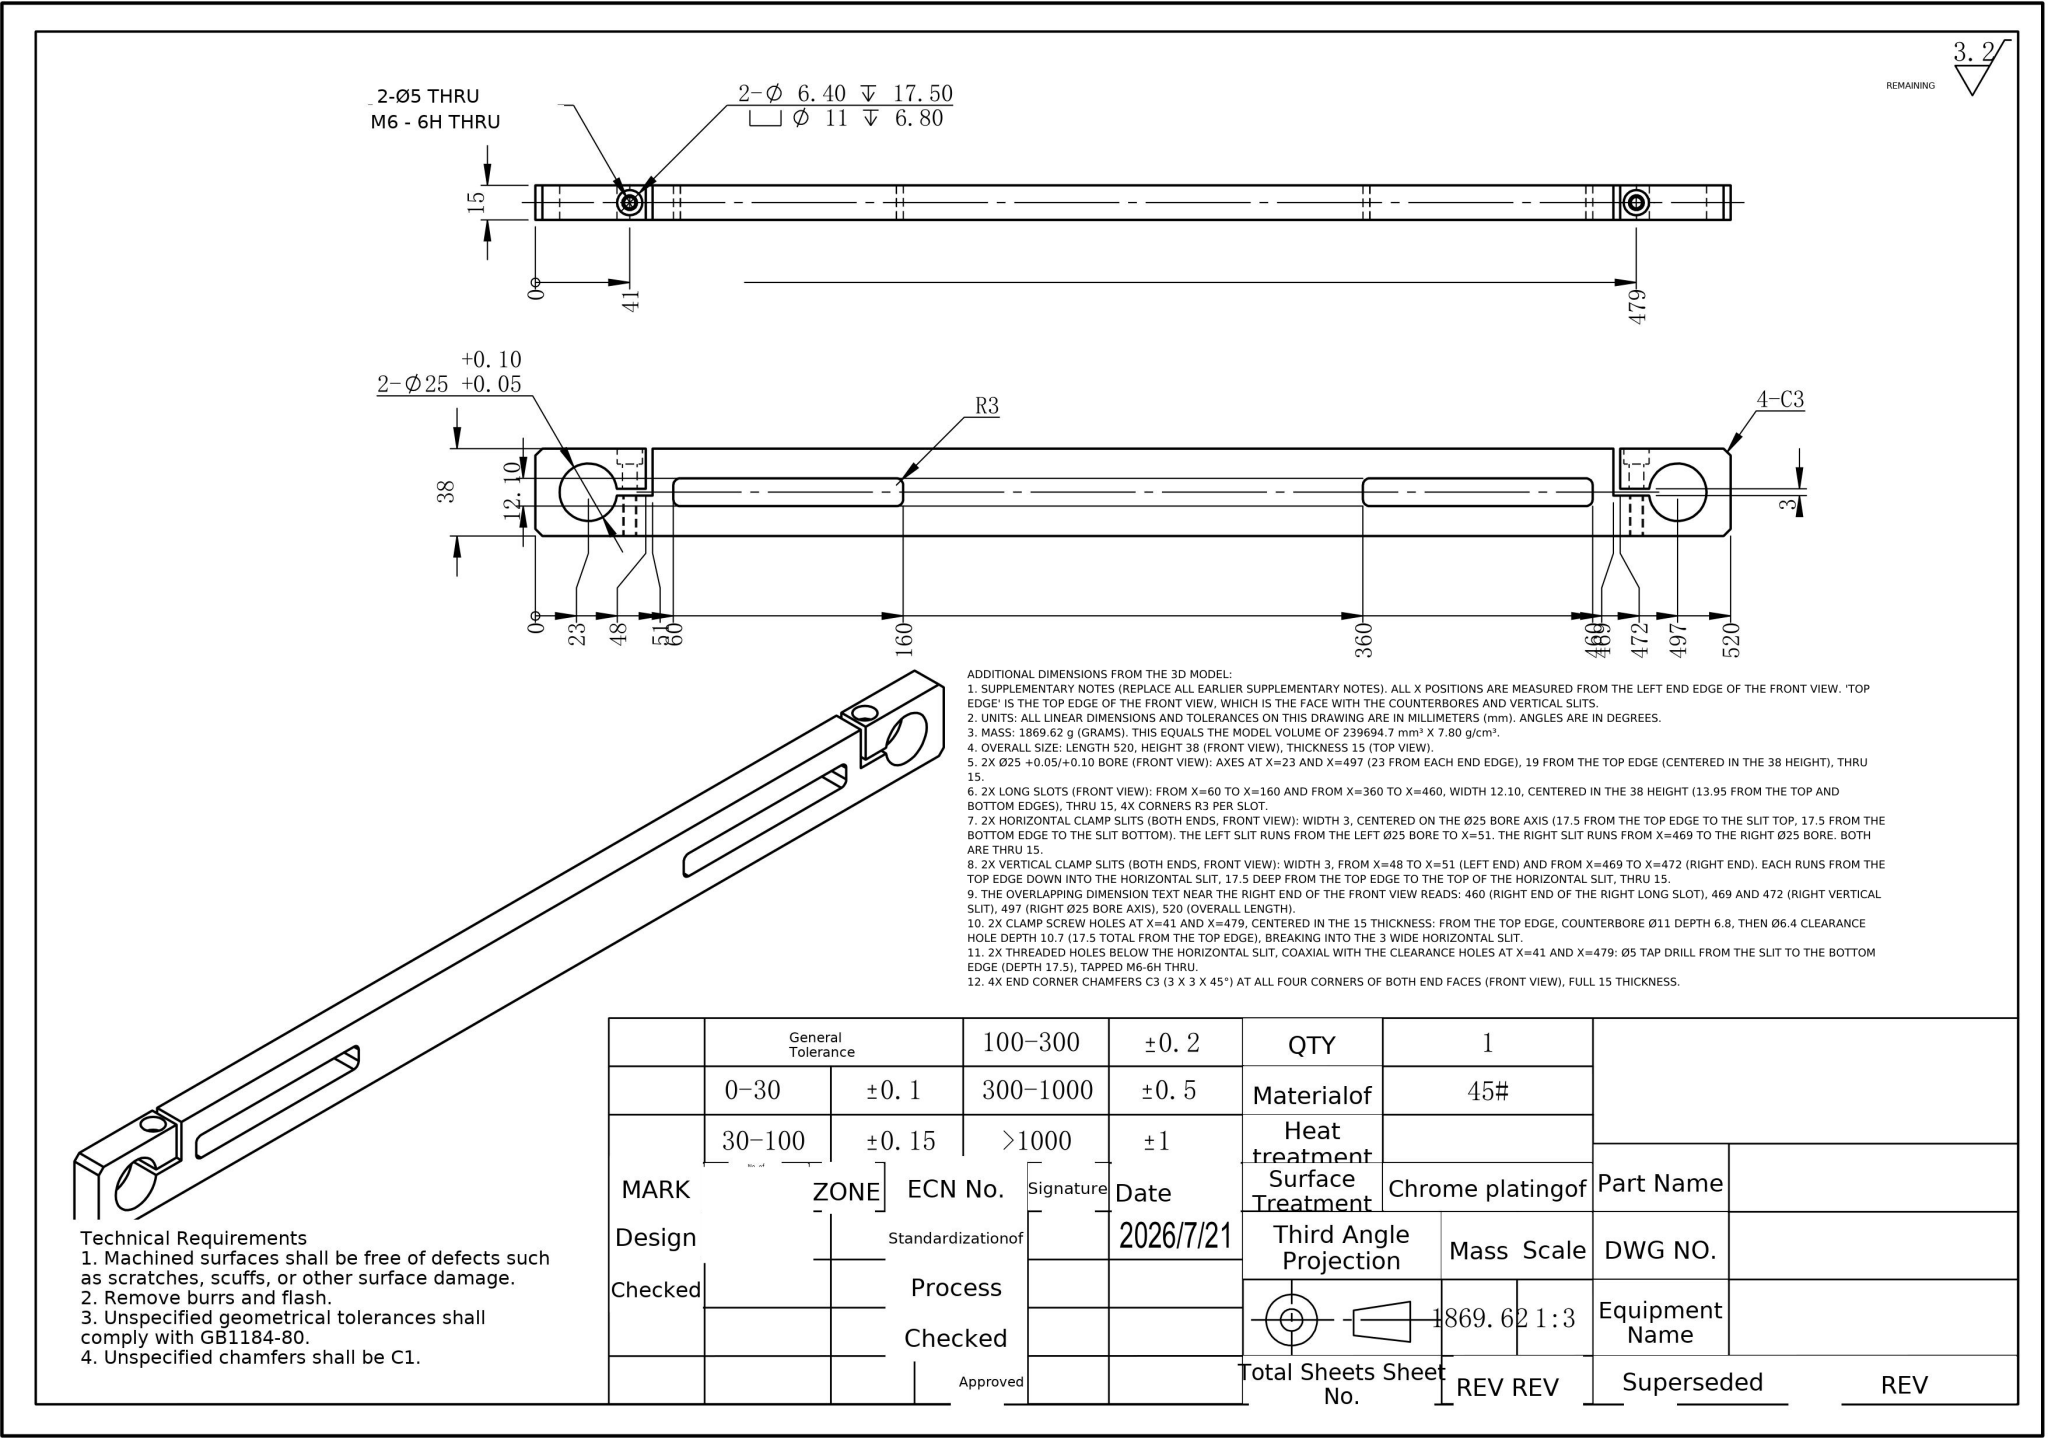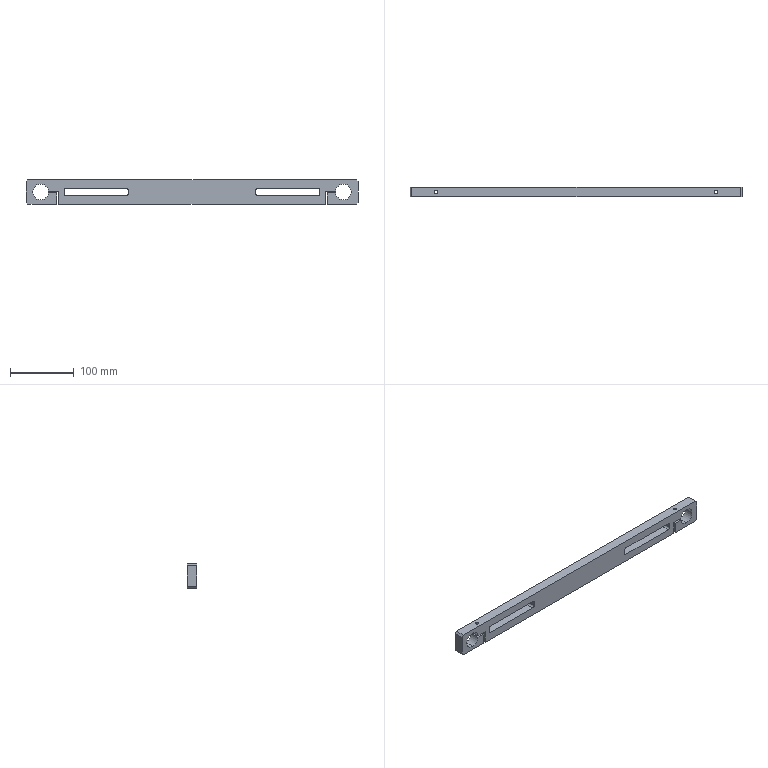Part | NX | mm | 1 solid | 56 faces | box 520 x 15 x 38 mm | volume 239695 mm3 | plane 30 | cylinder 26 | commonest cylinder face diameters 6 x8 25 x6 5 x4 11 x4 6.4 x4